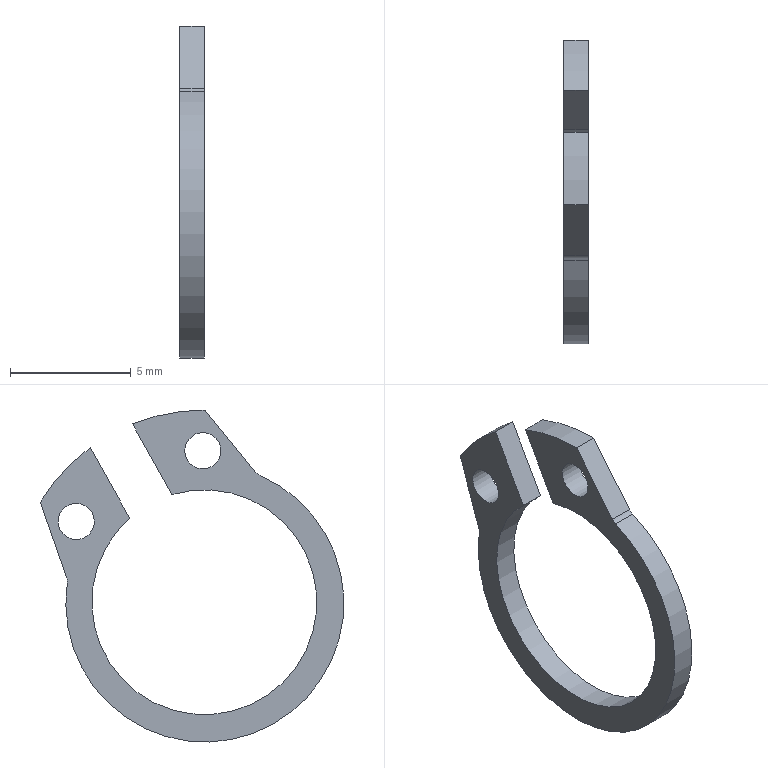Component | NX | RETAINING_RING | 1 solid | 14 faces | box 1 x 12.55 x 13.73 mm | volume 46 mm3 | cylinder 8 | plane 6 | commonest cylinder face diameters 15.9 x2 1.5 x2 1 x2 11.5 x1 9.3 x1
STEP:
#1=CARTESIAN_POINT('',(0.,0.,0.));
#2=DIRECTION('',(0.,0.,1.));
#3=DIRECTION('',(1.,0.,0.));
#4=AXIS2_PLACEMENT_3D('',#1,#2,#3);
#5=CARTESIAN_POINT('',(19.707,5.692,-145.299));
#6=VERTEX_POINT('',#5);
#7=CARTESIAN_POINT('',(19.707,-2.293,-140.838));
#8=VERTEX_POINT('',#7);
#9=CARTESIAN_POINT('',(19.707,0.,-146.111));
#10=DIRECTION('',(-1.,0.,0.));
#11=DIRECTION('',(0.,-0.873,0.4877));
#12=AXIS2_PLACEMENT_3D('',#9,#10,#11);
#13=CIRCLE('',#12,5.75);
#14=CARTESIAN_POINT('',(19.707,0.,-146.111));
#15=DIRECTION('',(-1.,0.,0.));
#16=DIRECTION('',(0.,0.873,-0.4877));
#17=AXIS2_PLACEMENT_3D('',#14,#15,#16);
#18=CYLINDRICAL_SURFACE('',#17,5.75);
#19=CARTESIAN_POINT('',(-3.142,0.));
#20=DIRECTION('',(1.,0.));
#21=VECTOR('',#20,1.);
#22=LINE('',#19,#21);
#23=(GEOMETRIC_REPRESENTATION_CONTEXT(2)PARAMETRIC_REPRESENTATION_CONTEXT()REPRESENTATION_CONTEXT('',''));
#24=DEFINITIONAL_REPRESENTATION('',(#22),#23);
#25=PCURVE('',#18,#24);
#26=CARTESIAN_POINT('',(19.707,0.,-146.111));
#27=DIRECTION('',(-1.,0.,0.));
#28=DIRECTION('',(0.,0.873,-0.4877));
#29=AXIS2_PLACEMENT_3D('',#26,#27,#28);
#30=PLANE('',#29);
#31=CARTESIAN_POINT('',(0.,0.));
#32=DIRECTION('',(-1.,0.));
#33=AXIS2_PLACEMENT_2D('',#31,#32);
#34=CIRCLE('',#33,5.75);
#35=(GEOMETRIC_REPRESENTATION_CONTEXT(2)PARAMETRIC_REPRESENTATION_CONTEXT()REPRESENTATION_CONTEXT('',''));
#36=DEFINITIONAL_REPRESENTATION('',(#34),#35);
#37=PCURVE('',#30,#36);
#38=SURFACE_CURVE('',#13,(#25,#37),.PCURVE_S1.);
#39=EDGE_CURVE('',#6,#8,#38,.T.);
#40=ORIENTED_EDGE('',*,*,#39,.T.);
#41=CARTESIAN_POINT('',(18.707,-2.293,-140.838));
#42=VERTEX_POINT('',#41);
#43=CARTESIAN_POINT('',(19.707,-2.293,-140.838));
#44=DIRECTION('',(-1.,0.,0.));
#45=VECTOR('',#44,1.);
#46=LINE('',#43,#45);
#47=CARTESIAN_POINT('',(3.793,0.));
#48=DIRECTION('',(0.,1.));
#49=VECTOR('',#48,1.);
#50=LINE('',#47,#49);
#51=(GEOMETRIC_REPRESENTATION_CONTEXT(2)PARAMETRIC_REPRESENTATION_CONTEXT()REPRESENTATION_CONTEXT('',''));
#52=DEFINITIONAL_REPRESENTATION('',(#50),#51);
#53=PCURVE('',#18,#52);
#54=CARTESIAN_POINT('',(19.707,-2.492,-140.38));
#55=DIRECTION('',(-1.,0.,0.));
#56=DIRECTION('',(0.,0.873,-0.4877));
#57=AXIS2_PLACEMENT_3D('',#54,#55,#56);
#58=CYLINDRICAL_SURFACE('',#57,0.5);
#59=CARTESIAN_POINT('',(0.6512,0.));
#60=DIRECTION('',(0.,1.));
#61=VECTOR('',#60,1.);
#62=LINE('',#59,#61);
#63=(GEOMETRIC_REPRESENTATION_CONTEXT(2)PARAMETRIC_REPRESENTATION_CONTEXT()REPRESENTATION_CONTEXT('',''));
#64=DEFINITIONAL_REPRESENTATION('',(#62),#63);
#65=PCURVE('',#58,#64);
#66=SURFACE_CURVE('',#46,(#53,#65),.PCURVE_S1.);
#67=EDGE_CURVE('',#8,#42,#66,.T.);
#68=ORIENTED_EDGE('',*,*,#67,.T.);
#69=CARTESIAN_POINT('',(18.707,5.692,-145.299));
#70=VERTEX_POINT('',#69);
#71=CARTESIAN_POINT('',(18.707,0.,-146.111));
#72=DIRECTION('',(-1.,0.,0.));
#73=DIRECTION('',(0.,-0.873,0.4877));
#74=AXIS2_PLACEMENT_3D('',#71,#72,#73);
#75=CIRCLE('',#74,5.75);
#76=CARTESIAN_POINT('',(-3.142,1.));
#77=DIRECTION('',(1.,0.));
#78=VECTOR('',#77,1.);
#79=LINE('',#76,#78);
#80=(GEOMETRIC_REPRESENTATION_CONTEXT(2)PARAMETRIC_REPRESENTATION_CONTEXT()REPRESENTATION_CONTEXT('',''));
#81=DEFINITIONAL_REPRESENTATION('',(#79),#80);
#82=PCURVE('',#18,#81);
#83=CARTESIAN_POINT('',(18.707,0.,-146.111));
#84=DIRECTION('',(-1.,0.,0.));
#85=DIRECTION('',(0.,0.873,-0.4877));
#86=AXIS2_PLACEMENT_3D('',#83,#84,#85);
#87=PLANE('',#86);
#88=CARTESIAN_POINT('',(0.,0.));
#89=DIRECTION('',(-1.,0.));
#90=AXIS2_PLACEMENT_2D('',#88,#89);
#91=CIRCLE('',#90,5.75);
#92=(GEOMETRIC_REPRESENTATION_CONTEXT(2)PARAMETRIC_REPRESENTATION_CONTEXT()REPRESENTATION_CONTEXT('',''));
#93=DEFINITIONAL_REPRESENTATION('',(#91),#92);
#94=PCURVE('',#87,#93);
#95=SURFACE_CURVE('',#75,(#82,#94),.PCURVE_S1.);
#96=EDGE_CURVE('',#70,#42,#95,.T.);
#97=ORIENTED_EDGE('',*,*,#96,.F.);
#98=CARTESIAN_POINT('',(19.707,5.692,-145.299));
#99=DIRECTION('',(1.,0.,0.));
#100=VECTOR('',#99,1.);
#101=LINE('',#98,#100);
#102=CARTESIAN_POINT('',(-0.6512,0.));
#103=DIRECTION('',(0.,-1.));
#104=VECTOR('',#103,1.);
#105=LINE('',#102,#104);
#106=(GEOMETRIC_REPRESENTATION_CONTEXT(2)PARAMETRIC_REPRESENTATION_CONTEXT()REPRESENTATION_CONTEXT('',''));
#107=DEFINITIONAL_REPRESENTATION('',(#105),#106);
#108=PCURVE('',#18,#107);
#109=CARTESIAN_POINT('',(19.707,6.187,-145.228));
#110=DIRECTION('',(-1.,0.,0.));
#111=DIRECTION('',(0.,0.873,-0.4877));
#112=AXIS2_PLACEMENT_3D('',#109,#110,#111);
#113=CYLINDRICAL_SURFACE('',#112,0.5);
#114=CARTESIAN_POINT('',(2.49,0.));
#115=DIRECTION('',(0.,-1.));
#116=VECTOR('',#115,1.);
#117=LINE('',#114,#116);
#118=(GEOMETRIC_REPRESENTATION_CONTEXT(2)PARAMETRIC_REPRESENTATION_CONTEXT()REPRESENTATION_CONTEXT('',''));
#119=DEFINITIONAL_REPRESENTATION('',(#117),#118);
#120=PCURVE('',#113,#119);
#121=SURFACE_CURVE('',#101,(#108,#120),.PCURVE_S1.);
#122=EDGE_CURVE('',#70,#6,#121,.T.);
#123=ORIENTED_EDGE('',*,*,#122,.T.);
#124=EDGE_LOOP('',(#40,#68,#97,#123));
#125=FACE_BOUND('',#124,.T.);
#126=ADVANCED_FACE('',(#125),#18,.T.);
#127=CARTESIAN_POINT('',(18.707,-2.105,-140.696));
#128=VERTEX_POINT('',#127);
#129=CARTESIAN_POINT('',(18.707,-0.01008,-138.126));
#130=VERTEX_POINT('',#129);
#131=CARTESIAN_POINT('',(18.707,-2.183,-140.792));
#132=DIRECTION('',(0.,0.6319,0.7751));
#133=VECTOR('',#132,1.);
#134=LINE('',#131,#133);
#135=CARTESIAN_POINT('',(19.707,-2.183,-140.792));
#136=DIRECTION('',(0.,-0.7751,0.6319));
#137=DIRECTION('',(0.,-0.6319,-0.7751));
#138=AXIS2_PLACEMENT_3D('',#135,#136,#137);
#139=PLANE('',#138);
#140=CARTESIAN_POINT('',(0.,-1.));
#141=DIRECTION('',(-1.,0.));
#142=VECTOR('',#141,1.);
#143=LINE('',#140,#142);
#144=(GEOMETRIC_REPRESENTATION_CONTEXT(2)PARAMETRIC_REPRESENTATION_CONTEXT()REPRESENTATION_CONTEXT('',''));
#145=DEFINITIONAL_REPRESENTATION('',(#143),#144);
#146=PCURVE('',#139,#145);
#147=CARTESIAN_POINT('',(-4.5,-3.579));
#148=DIRECTION('',(0.1736,-0.9848));
#149=VECTOR('',#148,1.);
#150=LINE('',#147,#149);
#151=(GEOMETRIC_REPRESENTATION_CONTEXT(2)PARAMETRIC_REPRESENTATION_CONTEXT()REPRESENTATION_CONTEXT('',''));
#152=DEFINITIONAL_REPRESENTATION('',(#150),#151);
#153=PCURVE('',#87,#152);
#154=SURFACE_CURVE('',#134,(#146,#153),.PCURVE_S1.);
#155=EDGE_CURVE('',#128,#130,#154,.T.);
#156=ORIENTED_EDGE('',*,*,#155,.F.);
#157=CARTESIAN_POINT('',(19.707,-2.105,-140.696));
#158=VERTEX_POINT('',#157);
#159=CARTESIAN_POINT('',(19.707,-2.105,-140.696));
#160=DIRECTION('',(1.,0.,0.));
#161=VECTOR('',#160,1.);
#162=LINE('',#159,#161);
#163=CARTESIAN_POINT('',(-0.1242,0.));
#164=DIRECTION('',(0.,1.));
#165=VECTOR('',#164,1.);
#166=LINE('',#163,#165);
#167=(GEOMETRIC_REPRESENTATION_CONTEXT(2)PARAMETRIC_REPRESENTATION_CONTEXT()REPRESENTATION_CONTEXT('',''));
#168=DEFINITIONAL_REPRESENTATION('',(#166),#167);
#169=PCURVE('',#139,#168);
#170=CARTESIAN_POINT('',(0.1745,0.));
#171=DIRECTION('',(0.,-1.));
#172=VECTOR('',#171,1.);
#173=LINE('',#170,#172);
#174=(GEOMETRIC_REPRESENTATION_CONTEXT(2)PARAMETRIC_REPRESENTATION_CONTEXT()REPRESENTATION_CONTEXT('',''));
#175=DEFINITIONAL_REPRESENTATION('',(#173),#174);
#176=PCURVE('',#58,#175);
#177=SURFACE_CURVE('',#162,(#169,#176),.PCURVE_S1.);
#178=EDGE_CURVE('',#128,#158,#177,.T.);
#179=ORIENTED_EDGE('',*,*,#178,.T.);
#180=CARTESIAN_POINT('',(19.707,-0.01008,-138.126));
#181=VERTEX_POINT('',#180);
#182=CARTESIAN_POINT('',(19.707,-2.183,-140.792));
#183=DIRECTION('',(0.,0.6319,0.7751));
#184=VECTOR('',#183,1.);
#185=LINE('',#182,#184);
#186=CARTESIAN_POINT('',(0.,0.));
#187=DIRECTION('',(-1.,0.));
#188=VECTOR('',#187,1.);
#189=LINE('',#186,#188);
#190=(GEOMETRIC_REPRESENTATION_CONTEXT(2)PARAMETRIC_REPRESENTATION_CONTEXT()REPRESENTATION_CONTEXT('',''));
#191=DEFINITIONAL_REPRESENTATION('',(#189),#190);
#192=PCURVE('',#139,#191);
#193=CARTESIAN_POINT('',(-4.5,-3.579));
#194=DIRECTION('',(0.1736,-0.9848));
#195=VECTOR('',#194,1.);
#196=LINE('',#193,#195);
#197=(GEOMETRIC_REPRESENTATION_CONTEXT(2)PARAMETRIC_REPRESENTATION_CONTEXT()REPRESENTATION_CONTEXT('',''));
#198=DEFINITIONAL_REPRESENTATION('',(#196),#197);
#199=PCURVE('',#30,#198);
#200=SURFACE_CURVE('',#185,(#192,#199),.PCURVE_S1.);
#201=EDGE_CURVE('',#158,#181,#200,.T.);
#202=ORIENTED_EDGE('',*,*,#201,.T.);
#203=CARTESIAN_POINT('',(19.707,-0.01008,-138.126));
#204=DIRECTION('',(-1.,0.,0.));
#205=VECTOR('',#204,1.);
#206=LINE('',#203,#205);
#207=CARTESIAN_POINT('',(-3.439,0.));
#208=DIRECTION('',(0.,-1.));
#209=VECTOR('',#208,1.);
#210=LINE('',#207,#209);
#211=(GEOMETRIC_REPRESENTATION_CONTEXT(2)PARAMETRIC_REPRESENTATION_CONTEXT()REPRESENTATION_CONTEXT('',''));
#212=DEFINITIONAL_REPRESENTATION('',(#210),#211);
#213=PCURVE('',#139,#212);
#214=CARTESIAN_POINT('',(19.707,0.01951,-146.076));
#215=DIRECTION('',(-1.,0.,0.));
#216=DIRECTION('',(0.,0.873,-0.4877));
#217=AXIS2_PLACEMENT_3D('',#214,#215,#216);
#218=CYLINDRICAL_SURFACE('',#217,7.95);
#219=CARTESIAN_POINT('',(4.199,0.));
#220=DIRECTION('',(0.,1.));
#221=VECTOR('',#220,1.);
#222=LINE('',#219,#221);
#223=(GEOMETRIC_REPRESENTATION_CONTEXT(2)PARAMETRIC_REPRESENTATION_CONTEXT()REPRESENTATION_CONTEXT('',''));
#224=DEFINITIONAL_REPRESENTATION('',(#222),#223);
#225=PCURVE('',#218,#224);
#226=SURFACE_CURVE('',#206,(#213,#225),.PCURVE_S1.);
#227=EDGE_CURVE('',#181,#130,#226,.T.);
#228=ORIENTED_EDGE('',*,*,#227,.T.);
#229=EDGE_LOOP('',(#156,#179,#202,#228));
#230=FACE_BOUND('',#229,.T.);
#231=ADVANCED_FACE('',(#230),#139,.T.);
#232=CARTESIAN_POINT('',(18.707,2.993,-138.703));
#233=VERTEX_POINT('',#232);
#234=CARTESIAN_POINT('',(18.707,0.01951,-146.076));
#235=DIRECTION('',(-1.,0.,0.));
#236=DIRECTION('',(0.,-0.873,0.4877));
#237=AXIS2_PLACEMENT_3D('',#234,#235,#236);
#238=CIRCLE('',#237,7.95);
#239=CARTESIAN_POINT('',(3.142,1.));
#240=DIRECTION('',(1.,0.));
#241=VECTOR('',#240,1.);
#242=LINE('',#239,#241);
#243=(GEOMETRIC_REPRESENTATION_CONTEXT(2)PARAMETRIC_REPRESENTATION_CONTEXT()REPRESENTATION_CONTEXT('',''));
#244=DEFINITIONAL_REPRESENTATION('',(#242),#243);
#245=PCURVE('',#218,#244);
#246=CARTESIAN_POINT('',(-0.,-0.04));
#247=DIRECTION('',(-1.,0.));
#248=AXIS2_PLACEMENT_2D('',#246,#247);
#249=CIRCLE('',#248,7.95);
#250=(GEOMETRIC_REPRESENTATION_CONTEXT(2)PARAMETRIC_REPRESENTATION_CONTEXT()REPRESENTATION_CONTEXT('',''));
#251=DEFINITIONAL_REPRESENTATION('',(#249),#250);
#252=PCURVE('',#87,#251);
#253=SURFACE_CURVE('',#238,(#245,#252),.PCURVE_S1.);
#254=EDGE_CURVE('',#130,#233,#253,.T.);
#255=ORIENTED_EDGE('',*,*,#254,.F.);
#256=ORIENTED_EDGE('',*,*,#227,.F.);
#257=CARTESIAN_POINT('',(19.707,2.993,-138.703));
#258=VERTEX_POINT('',#257);
#259=CARTESIAN_POINT('',(19.707,0.01951,-146.076));
#260=DIRECTION('',(-1.,0.,0.));
#261=DIRECTION('',(0.,-0.873,0.4877));
#262=AXIS2_PLACEMENT_3D('',#259,#260,#261);
#263=CIRCLE('',#262,7.95);
#264=CARTESIAN_POINT('',(3.142,0.));
#265=DIRECTION('',(1.,0.));
#266=VECTOR('',#265,1.);
#267=LINE('',#264,#266);
#268=(GEOMETRIC_REPRESENTATION_CONTEXT(2)PARAMETRIC_REPRESENTATION_CONTEXT()REPRESENTATION_CONTEXT('',''));
#269=DEFINITIONAL_REPRESENTATION('',(#267),#268);
#270=PCURVE('',#218,#269);
#271=CARTESIAN_POINT('',(-0.,-0.04));
#272=DIRECTION('',(-1.,0.));
#273=AXIS2_PLACEMENT_2D('',#271,#272);
#274=CIRCLE('',#273,7.95);
#275=(GEOMETRIC_REPRESENTATION_CONTEXT(2)PARAMETRIC_REPRESENTATION_CONTEXT()REPRESENTATION_CONTEXT('',''));
#276=DEFINITIONAL_REPRESENTATION('',(#274),#275);
#277=PCURVE('',#30,#276);
#278=SURFACE_CURVE('',#263,(#270,#277),.PCURVE_S1.);
#279=EDGE_CURVE('',#181,#258,#278,.T.);
#280=ORIENTED_EDGE('',*,*,#279,.T.);
#281=CARTESIAN_POINT('',(19.707,2.993,-138.703));
#282=DIRECTION('',(-1.,0.,0.));
#283=VECTOR('',#282,1.);
#284=LINE('',#281,#283);
#285=CARTESIAN_POINT('',(4.586,0.));
#286=DIRECTION('',(0.,1.));
#287=VECTOR('',#286,1.);
#288=LINE('',#285,#287);
#289=(GEOMETRIC_REPRESENTATION_CONTEXT(2)PARAMETRIC_REPRESENTATION_CONTEXT()REPRESENTATION_CONTEXT('',''));
#290=DEFINITIONAL_REPRESENTATION('',(#288),#289);
#291=PCURVE('',#218,#290);
#292=CARTESIAN_POINT('',(19.707,2.993,-138.703));
#293=DIRECTION('',(0.,0.873,-0.4877));
#294=DIRECTION('',(0.,0.4877,0.873));
#295=AXIS2_PLACEMENT_3D('',#292,#293,#294);
#296=PLANE('',#295);
#297=CARTESIAN_POINT('',(0.,0.));
#298=DIRECTION('',(0.,-1.));
#299=VECTOR('',#298,1.);
#300=LINE('',#297,#299);
#301=(GEOMETRIC_REPRESENTATION_CONTEXT(2)PARAMETRIC_REPRESENTATION_CONTEXT()REPRESENTATION_CONTEXT('',''));
#302=DEFINITIONAL_REPRESENTATION('',(#300),#301);
#303=PCURVE('',#296,#302);
#304=SURFACE_CURVE('',#284,(#291,#303),.PCURVE_S1.);
#305=EDGE_CURVE('',#258,#233,#304,.T.);
#306=ORIENTED_EDGE('',*,*,#305,.T.);
#307=EDGE_LOOP('',(#255,#256,#280,#306));
#308=FACE_BOUND('',#307,.T.);
#309=ADVANCED_FACE('',(#308),#218,.T.);
#310=CARTESIAN_POINT('',(18.707,1.361,-141.624));
#311=VERTEX_POINT('',#310);
#312=CARTESIAN_POINT('',(18.707,2.993,-138.703));
#313=DIRECTION('',(0.,-0.4877,-0.873));
#314=VECTOR('',#313,1.);
#315=LINE('',#312,#314);
#316=CARTESIAN_POINT('',(0.,-1.));
#317=DIRECTION('',(-1.,0.));
#318=VECTOR('',#317,1.);
#319=LINE('',#316,#318);
#320=(GEOMETRIC_REPRESENTATION_CONTEXT(2)PARAMETRIC_REPRESENTATION_CONTEXT()REPRESENTATION_CONTEXT('',''));
#321=DEFINITIONAL_REPRESENTATION('',(#319),#320);
#322=PCURVE('',#296,#321);
#323=CARTESIAN_POINT('',(-1.,-7.927));
#324=DIRECTION('',(0.,1.));
#325=VECTOR('',#324,1.);
#326=LINE('',#323,#325);
#327=(GEOMETRIC_REPRESENTATION_CONTEXT(2)PARAMETRIC_REPRESENTATION_CONTEXT()REPRESENTATION_CONTEXT('',''));
#328=DEFINITIONAL_REPRESENTATION('',(#326),#327);
#329=PCURVE('',#87,#328);
#330=SURFACE_CURVE('',#315,(#322,#329),.PCURVE_S1.);
#331=EDGE_CURVE('',#233,#311,#330,.T.);
#332=ORIENTED_EDGE('',*,*,#331,.F.);
#333=ORIENTED_EDGE('',*,*,#305,.F.);
#334=CARTESIAN_POINT('',(19.707,1.361,-141.624));
#335=VERTEX_POINT('',#334);
#336=CARTESIAN_POINT('',(19.707,2.993,-138.703));
#337=DIRECTION('',(0.,-0.4877,-0.873));
#338=VECTOR('',#337,1.);
#339=LINE('',#336,#338);
#340=CARTESIAN_POINT('',(0.,0.));
#341=DIRECTION('',(-1.,0.));
#342=VECTOR('',#341,1.);
#343=LINE('',#340,#342);
#344=(GEOMETRIC_REPRESENTATION_CONTEXT(2)PARAMETRIC_REPRESENTATION_CONTEXT()REPRESENTATION_CONTEXT('',''));
#345=DEFINITIONAL_REPRESENTATION('',(#343),#344);
#346=PCURVE('',#296,#345);
#347=CARTESIAN_POINT('',(-1.,-7.927));
#348=DIRECTION('',(0.,1.));
#349=VECTOR('',#348,1.);
#350=LINE('',#347,#349);
#351=(GEOMETRIC_REPRESENTATION_CONTEXT(2)PARAMETRIC_REPRESENTATION_CONTEXT()REPRESENTATION_CONTEXT('',''));
#352=DEFINITIONAL_REPRESENTATION('',(#350),#351);
#353=PCURVE('',#30,#352);
#354=SURFACE_CURVE('',#339,(#346,#353),.PCURVE_S1.);
#355=EDGE_CURVE('',#258,#335,#354,.T.);
#356=ORIENTED_EDGE('',*,*,#355,.T.);
#357=CARTESIAN_POINT('',(19.707,1.361,-141.624));
#358=DIRECTION('',(-1.,0.,0.));
#359=VECTOR('',#358,1.);
#360=LINE('',#357,#359);
#361=CARTESIAN_POINT('',(-3.346,0.));
#362=DIRECTION('',(0.,-1.));
#363=VECTOR('',#362,1.);
#364=LINE('',#361,#363);
#365=(GEOMETRIC_REPRESENTATION_CONTEXT(2)PARAMETRIC_REPRESENTATION_CONTEXT()REPRESENTATION_CONTEXT('',''));
#366=DEFINITIONAL_REPRESENTATION('',(#364),#365);
#367=PCURVE('',#296,#366);
#368=CARTESIAN_POINT('',(19.707,0.01951,-146.076));
#369=DIRECTION('',(-1.,0.,0.));
#370=DIRECTION('',(0.,0.873,-0.4877));
#371=AXIS2_PLACEMENT_3D('',#368,#369,#370);
#372=CYLINDRICAL_SURFACE('',#371,4.65);
#373=CARTESIAN_POINT('',(4.496,0.));
#374=DIRECTION('',(0.,1.));
#375=VECTOR('',#374,1.);
#376=LINE('',#373,#375);
#377=(GEOMETRIC_REPRESENTATION_CONTEXT(2)PARAMETRIC_REPRESENTATION_CONTEXT()REPRESENTATION_CONTEXT('',''));
#378=DEFINITIONAL_REPRESENTATION('',(#376),#377);
#379=PCURVE('',#372,#378);
#380=SURFACE_CURVE('',#360,(#367,#379),.PCURVE_S1.);
#381=EDGE_CURVE('',#335,#311,#380,.T.);
#382=ORIENTED_EDGE('',*,*,#381,.T.);
#383=EDGE_LOOP('',(#332,#333,#356,#382));
#384=FACE_BOUND('',#383,.T.);
#385=ADVANCED_FACE('',(#384),#296,.T.);
#386=CARTESIAN_POINT('',(19.707,3.107,-142.599));
#387=VERTEX_POINT('',#386);
#388=CARTESIAN_POINT('',(18.707,3.107,-142.599));
#389=VERTEX_POINT('',#388);
#390=CARTESIAN_POINT('',(19.707,3.107,-142.599));
#391=DIRECTION('',(-1.,0.,0.));
#392=VECTOR('',#391,1.);
#393=LINE('',#390,#392);
#394=CARTESIAN_POINT('',(-1.354,0.));
#395=DIRECTION('',(0.,1.));
#396=VECTOR('',#395,1.);
#397=LINE('',#394,#396);
#398=(GEOMETRIC_REPRESENTATION_CONTEXT(2)PARAMETRIC_REPRESENTATION_CONTEXT()REPRESENTATION_CONTEXT('',''));
#399=DEFINITIONAL_REPRESENTATION('',(#397),#398);
#400=PCURVE('',#372,#399);
#401=CARTESIAN_POINT('',(19.707,3.107,-142.599));
#402=DIRECTION('',(0.,-0.873,0.4877));
#403=DIRECTION('',(0.,-0.4877,-0.873));
#404=AXIS2_PLACEMENT_3D('',#401,#402,#403);
#405=PLANE('',#404);
#406=CARTESIAN_POINT('',(0.,0.));
#407=DIRECTION('',(0.,-1.));
#408=VECTOR('',#407,1.);
#409=LINE('',#406,#408);
#410=(GEOMETRIC_REPRESENTATION_CONTEXT(2)PARAMETRIC_REPRESENTATION_CONTEXT()REPRESENTATION_CONTEXT('',''));
#411=DEFINITIONAL_REPRESENTATION('',(#409),#410);
#412=PCURVE('',#405,#411);
#413=SURFACE_CURVE('',#393,(#400,#412),.PCURVE_S1.);
#414=EDGE_CURVE('',#387,#389,#413,.T.);
#415=ORIENTED_EDGE('',*,*,#414,.F.);
#416=CARTESIAN_POINT('',(19.707,0.01951,-146.076));
#417=DIRECTION('',(1.,0.,0.));
#418=DIRECTION('',(0.,-0.873,0.4877));
#419=AXIS2_PLACEMENT_3D('',#416,#417,#418);
#420=CIRCLE('',#419,4.65);
#421=CARTESIAN_POINT('',(9.425,0.));
#422=DIRECTION('',(-1.,0.));
#423=VECTOR('',#422,1.);
#424=LINE('',#421,#423);
#425=(GEOMETRIC_REPRESENTATION_CONTEXT(2)PARAMETRIC_REPRESENTATION_CONTEXT()REPRESENTATION_CONTEXT('',''));
#426=DEFINITIONAL_REPRESENTATION('',(#424),#425);
#427=PCURVE('',#372,#426);
#428=CARTESIAN_POINT('',(-4.65,-0.04));
#429=CARTESIAN_POINT('',(-4.65,8.014));
#430=CARTESIAN_POINT('',(2.325,3.987));
#431=CARTESIAN_POINT('',(9.3,-0.04));
#432=CARTESIAN_POINT('',(2.325,-4.067));
#433=CARTESIAN_POINT('',(-4.65,-8.094));
#434=CARTESIAN_POINT('',(-4.65,-0.04));
#435=(BOUNDED_CURVE()B_SPLINE_CURVE(2,(#428,#429,#430,#431,#432,#433,#434),.UNSPECIFIED.,.T.,.F.)B_SPLINE_CURVE_WITH_KNOTS((1,2,2,2,2,1),(-2.094,0.,2.094,4.189,6.283,8.378),.UNSPECIFIED.)CURVE()GEOMETRIC_REPRESENTATION_ITEM()RATIONAL_B_SPLINE_CURVE((1.,0.5,1.,0.5,1.,0.5,1.))REPRESENTATION_ITEM(''));
#436=(GEOMETRIC_REPRESENTATION_CONTEXT(2)PARAMETRIC_REPRESENTATION_CONTEXT()REPRESENTATION_CONTEXT('',''));
#437=DEFINITIONAL_REPRESENTATION('',(#435),#436);
#438=PCURVE('',#30,#437);
#439=SURFACE_CURVE('',#420,(#427,#438),.PCURVE_S1.);
#440=EDGE_CURVE('',#335,#387,#439,.T.);
#441=ORIENTED_EDGE('',*,*,#440,.F.);
#442=ORIENTED_EDGE('',*,*,#381,.T.);
#443=CARTESIAN_POINT('',(18.707,0.01951,-146.076));
#444=DIRECTION('',(1.,0.,0.));
#445=DIRECTION('',(0.,-0.873,0.4877));
#446=AXIS2_PLACEMENT_3D('',#443,#444,#445);
#447=CIRCLE('',#446,4.65);
#448=CARTESIAN_POINT('',(9.425,1.));
#449=DIRECTION('',(-1.,0.));
#450=VECTOR('',#449,1.);
#451=LINE('',#448,#450);
#452=(GEOMETRIC_REPRESENTATION_CONTEXT(2)PARAMETRIC_REPRESENTATION_CONTEXT()REPRESENTATION_CONTEXT('',''));
#453=DEFINITIONAL_REPRESENTATION('',(#451),#452);
#454=PCURVE('',#372,#453);
#455=CARTESIAN_POINT('',(-4.65,-0.04));
#456=CARTESIAN_POINT('',(-4.65,8.014));
#457=CARTESIAN_POINT('',(2.325,3.987));
#458=CARTESIAN_POINT('',(9.3,-0.04));
#459=CARTESIAN_POINT('',(2.325,-4.067));
#460=CARTESIAN_POINT('',(-4.65,-8.094));
#461=CARTESIAN_POINT('',(-4.65,-0.04));
#462=(BOUNDED_CURVE()B_SPLINE_CURVE(2,(#455,#456,#457,#458,#459,#460,#461),.UNSPECIFIED.,.T.,.F.)B_SPLINE_CURVE_WITH_KNOTS((1,2,2,2,2,1),(-2.094,0.,2.094,4.189,6.283,8.378),.UNSPECIFIED.)CURVE()GEOMETRIC_REPRESENTATION_ITEM()RATIONAL_B_SPLINE_CURVE((1.,0.5,1.,0.5,1.,0.5,1.))REPRESENTATION_ITEM(''));
#463=(GEOMETRIC_REPRESENTATION_CONTEXT(2)PARAMETRIC_REPRESENTATION_CONTEXT()REPRESENTATION_CONTEXT('',''));
#464=DEFINITIONAL_REPRESENTATION('',(#462),#463);
#465=PCURVE('',#87,#464);
#466=SURFACE_CURVE('',#447,(#454,#465),.PCURVE_S1.);
#467=EDGE_CURVE('',#311,#389,#466,.T.);
#468=ORIENTED_EDGE('',*,*,#467,.T.);
#469=EDGE_LOOP('',(#415,#441,#442,#468));
#470=FACE_BOUND('',#469,.F.);
#471=ADVANCED_FACE('',(#470),#372,.F.);
#472=CARTESIAN_POINT('',(18.707,4.739,-139.679));
#473=VERTEX_POINT('',#472);
#474=CARTESIAN_POINT('',(18.707,3.107,-142.599));
#475=DIRECTION('',(0.,0.4877,0.873));
#476=VECTOR('',#475,1.);
#477=LINE('',#474,#476);
#478=CARTESIAN_POINT('',(0.,-1.));
#479=DIRECTION('',(-1.,0.));
#480=VECTOR('',#479,1.);
#481=LINE('',#478,#480);
#482=(GEOMETRIC_REPRESENTATION_CONTEXT(2)PARAMETRIC_REPRESENTATION_CONTEXT()REPRESENTATION_CONTEXT('',''));
#483=DEFINITIONAL_REPRESENTATION('',(#481),#482);
#484=PCURVE('',#405,#483);
#485=CARTESIAN_POINT('',(1.,-4.581));
#486=DIRECTION('',(0.,-1.));
#487=VECTOR('',#486,1.);
#488=LINE('',#485,#487);
#489=(GEOMETRIC_REPRESENTATION_CONTEXT(2)PARAMETRIC_REPRESENTATION_CONTEXT()REPRESENTATION_CONTEXT('',''));
#490=DEFINITIONAL_REPRESENTATION('',(#488),#489);
#491=PCURVE('',#87,#490);
#492=SURFACE_CURVE('',#477,(#484,#491),.PCURVE_S1.);
#493=EDGE_CURVE('',#389,#473,#492,.T.);
#494=ORIENTED_EDGE('',*,*,#493,.F.);
#495=ORIENTED_EDGE('',*,*,#414,.F.);
#496=CARTESIAN_POINT('',(19.707,4.739,-139.679));
#497=VERTEX_POINT('',#496);
#498=CARTESIAN_POINT('',(19.707,3.107,-142.599));
#499=DIRECTION('',(0.,0.4877,0.873));
#500=VECTOR('',#499,1.);
#501=LINE('',#498,#500);
#502=CARTESIAN_POINT('',(0.,0.));
#503=DIRECTION('',(-1.,0.));
#504=VECTOR('',#503,1.);
#505=LINE('',#502,#504);
#506=(GEOMETRIC_REPRESENTATION_CONTEXT(2)PARAMETRIC_REPRESENTATION_CONTEXT()REPRESENTATION_CONTEXT('',''));
#507=DEFINITIONAL_REPRESENTATION('',(#505),#506);
#508=PCURVE('',#405,#507);
#509=CARTESIAN_POINT('',(1.,-4.581));
#510=DIRECTION('',(0.,-1.));
#511=VECTOR('',#510,1.);
#512=LINE('',#509,#511);
#513=(GEOMETRIC_REPRESENTATION_CONTEXT(2)PARAMETRIC_REPRESENTATION_CONTEXT()REPRESENTATION_CONTEXT('',''));
#514=DEFINITIONAL_REPRESENTATION('',(#512),#513);
#515=PCURVE('',#30,#514);
#516=SURFACE_CURVE('',#501,(#508,#515),.PCURVE_S1.);
#517=EDGE_CURVE('',#387,#497,#516,.T.);
#518=ORIENTED_EDGE('',*,*,#517,.T.);
#519=CARTESIAN_POINT('',(19.707,4.739,-139.679));
#520=DIRECTION('',(-1.,0.,0.));
#521=VECTOR('',#520,1.);
#522=LINE('',#519,#521);
#523=CARTESIAN_POINT('',(-3.346,0.));
#524=DIRECTION('',(0.,-1.));
#525=VECTOR('',#524,1.);
#526=LINE('',#523,#525);
#527=(GEOMETRIC_REPRESENTATION_CONTEXT(2)PARAMETRIC_REPRESENTATION_CONTEXT()REPRESENTATION_CONTEXT('',''));
#528=DEFINITIONAL_REPRESENTATION('',(#526),#527);
#529=PCURVE('',#405,#528);
#530=CARTESIAN_POINT('',(19.707,0.01951,-146.076));
#531=DIRECTION('',(-1.,0.,0.));
#532=DIRECTION('',(0.,0.873,-0.4877));
#533=AXIS2_PLACEMENT_3D('',#530,#531,#532);
#534=CYLINDRICAL_SURFACE('',#533,7.95);
#535=CARTESIAN_POINT('',(4.839,0.));
#536=DIRECTION('',(0.,1.));
#537=VECTOR('',#536,1.);
#538=LINE('',#535,#537);
#539=(GEOMETRIC_REPRESENTATION_CONTEXT(2)PARAMETRIC_REPRESENTATION_CONTEXT()REPRESENTATION_CONTEXT('',''));
#540=DEFINITIONAL_REPRESENTATION('',(#538),#539);
#541=PCURVE('',#534,#540);
#542=SURFACE_CURVE('',#522,(#529,#541),.PCURVE_S1.);
#543=EDGE_CURVE('',#497,#473,#542,.T.);
#544=ORIENTED_EDGE('',*,*,#543,.T.);
#545=EDGE_LOOP('',(#494,#495,#518,#544));
#546=FACE_BOUND('',#545,.T.);
#547=ADVANCED_FACE('',(#546),#405,.T.);
#548=CARTESIAN_POINT('',(18.707,6.804,-141.933));
#549=VERTEX_POINT('',#548);
#550=CARTESIAN_POINT('',(18.707,0.01951,-146.076));
#551=DIRECTION('',(-1.,0.,0.));
#552=DIRECTION('',(0.,-0.873,0.4877));
#553=AXIS2_PLACEMENT_3D('',#550,#551,#552);
#554=CIRCLE('',#553,7.95);
#555=CARTESIAN_POINT('',(3.142,1.));
#556=DIRECTION('',(1.,0.));
#557=VECTOR('',#556,1.);
#558=LINE('',#555,#557);
#559=(GEOMETRIC_REPRESENTATION_CONTEXT(2)PARAMETRIC_REPRESENTATION_CONTEXT()REPRESENTATION_CONTEXT('',''));
#560=DEFINITIONAL_REPRESENTATION('',(#558),#559);
#561=PCURVE('',#534,#560);
#562=CARTESIAN_POINT('',(-0.,-0.04));
#563=DIRECTION('',(-1.,0.));
#564=AXIS2_PLACEMENT_2D('',#562,#563);
#565=CIRCLE('',#564,7.95);
#566=(GEOMETRIC_REPRESENTATION_CONTEXT(2)PARAMETRIC_REPRESENTATION_CONTEXT()REPRESENTATION_CONTEXT('',''));
#567=DEFINITIONAL_REPRESENTATION('',(#565),#566);
#568=PCURVE('',#87,#567);
#569=SURFACE_CURVE('',#554,(#561,#568),.PCURVE_S1.);
#570=EDGE_CURVE('',#473,#549,#569,.T.);
#571=ORIENTED_EDGE('',*,*,#570,.F.);
#572=ORIENTED_EDGE('',*,*,#543,.F.);
#573=CARTESIAN_POINT('',(19.707,6.804,-141.933));
#574=VERTEX_POINT('',#573);
#575=CARTESIAN_POINT('',(19.707,0.01951,-146.076));
#576=DIRECTION('',(-1.,0.,0.));
#577=DIRECTION('',(0.,-0.873,0.4877));
#578=AXIS2_PLACEMENT_3D('',#575,#576,#577);
#579=CIRCLE('',#578,7.95);
#580=CARTESIAN_POINT('',(3.142,0.));
#581=DIRECTION('',(1.,0.));
#582=VECTOR('',#581,1.);
#583=LINE('',#580,#582);
#584=(GEOMETRIC_REPRESENTATION_CONTEXT(2)PARAMETRIC_REPRESENTATION_CONTEXT()REPRESENTATION_CONTEXT('',''));
#585=DEFINITIONAL_REPRESENTATION('',(#583),#584);
#586=PCURVE('',#534,#585);
#587=CARTESIAN_POINT('',(-0.,-0.04));
#588=DIRECTION('',(-1.,0.));
#589=AXIS2_PLACEMENT_2D('',#587,#588);
#590=CIRCLE('',#589,7.95);
#591=(GEOMETRIC_REPRESENTATION_CONTEXT(2)PARAMETRIC_REPRESENTATION_CONTEXT()REPRESENTATION_CONTEXT('',''));
#592=DEFINITIONAL_REPRESENTATION('',(#590),#591);
#593=PCURVE('',#30,#592);
#594=SURFACE_CURVE('',#579,(#586,#593),.PCURVE_S1.);
#595=EDGE_CURVE('',#497,#574,#594,.T.);
#596=ORIENTED_EDGE('',*,*,#595,.T.);
#597=CARTESIAN_POINT('',(19.707,6.804,-141.933));
#598=DIRECTION('',(-1.,0.,0.));
#599=VECTOR('',#598,1.);
#600=LINE('',#597,#599);
#601=CARTESIAN_POINT('',(5.226,0.));
#602=DIRECTION('',(0.,1.));
#603=VECTOR('',#602,1.);
#604=LINE('',#601,#603);
#605=(GEOMETRIC_REPRESENTATION_CONTEXT(2)PARAMETRIC_REPRESENTATION_CONTEXT()REPRESENTATION_CONTEXT('',''));
#606=DEFINITIONAL_REPRESENTATION('',(#604),#605);
#607=PCURVE('',#534,#606);
#608=CARTESIAN_POINT('',(19.707,6.804,-141.933));
#609=DIRECTION('',(0.,0.9444,-0.3287));
#610=DIRECTION('',(0.,0.3287,0.9444));
#611=AXIS2_PLACEMENT_3D('',#608,#609,#610);
#612=PLANE('',#611);
#613=CARTESIAN_POINT('',(-0.,0.));
#614=DIRECTION('',(0.,-1.));
#615=VECTOR('',#614,1.);
#616=LINE('',#613,#615);
#617=(GEOMETRIC_REPRESENTATION_CONTEXT(2)PARAMETRIC_REPRESENTATION_CONTEXT()REPRESENTATION_CONTEXT('',''));
#618=DEFINITIONAL_REPRESENTATION('',(#616),#617);
#619=PCURVE('',#612,#618);
#620=SURFACE_CURVE('',#600,(#607,#619),.PCURVE_S1.);
#621=EDGE_CURVE('',#574,#549,#620,.T.);
#622=ORIENTED_EDGE('',*,*,#621,.T.);
#623=EDGE_LOOP('',(#571,#572,#596,#622));
#624=FACE_BOUND('',#623,.T.);
#625=ADVANCED_FACE('',(#624),#534,.T.);
#626=CARTESIAN_POINT('',(19.707,0.7374,-140.177));
#627=VERTEX_POINT('',#626);
#628=CARTESIAN_POINT('',(19.707,0.08267,-139.812));
#629=DIRECTION('',(1.,0.,0.));
#630=DIRECTION('',(0.,0.873,-0.4877));
#631=AXIS2_PLACEMENT_3D('',#628,#629,#630);
#632=CIRCLE('',#631,0.75);
#633=CARTESIAN_POINT('',(19.707,0.08267,-139.812));
#634=DIRECTION('',(-1.,0.,0.));
#635=DIRECTION('',(0.,0.873,-0.4877));
#636=AXIS2_PLACEMENT_3D('',#633,#634,#635);
#637=CYLINDRICAL_SURFACE('',#636,0.75);
#638=CARTESIAN_POINT('',(6.283,0.));
#639=DIRECTION('',(-1.,0.));
#640=VECTOR('',#639,1.);
#641=LINE('',#638,#640);
#642=(GEOMETRIC_REPRESENTATION_CONTEXT(2)PARAMETRIC_REPRESENTATION_CONTEXT()REPRESENTATION_CONTEXT('',''));
#643=DEFINITIONAL_REPRESENTATION('',(#641),#642);
#644=PCURVE('',#637,#643);
#645=CARTESIAN_POINT('',(-2.25,-5.54));
#646=CARTESIAN_POINT('',(-2.25,-6.839));
#647=CARTESIAN_POINT('',(-3.375,-6.19));
#648=CARTESIAN_POINT('',(-4.5,-5.54));
#649=CARTESIAN_POINT('',(-3.375,-4.89));
#650=CARTESIAN_POINT('',(-2.25,-4.241));
#651=CARTESIAN_POINT('',(-2.25,-5.54));
#652=(BOUNDED_CURVE()B_SPLINE_CURVE(2,(#645,#646,#647,#648,#649,#650,#651),.UNSPECIFIED.,.T.,.F.)B_SPLINE_CURVE_WITH_KNOTS((1,2,2,2,2,1),(-2.094,0.,2.094,4.189,6.283,8.378),.UNSPECIFIED.)CURVE()GEOMETRIC_REPRESENTATION_ITEM()RATIONAL_B_SPLINE_CURVE((1.,0.5,1.,0.5,1.,0.5,1.))REPRESENTATION_ITEM(''));
#653=(GEOMETRIC_REPRESENTATION_CONTEXT(2)PARAMETRIC_REPRESENTATION_CONTEXT()REPRESENTATION_CONTEXT('',''));
#654=DEFINITIONAL_REPRESENTATION('',(#652),#653);
#655=PCURVE('',#30,#654);
#656=SURFACE_CURVE('',#632,(#644,#655),.PCURVE_S1.);
#657=EDGE_CURVE('',#627,#627,#656,.T.);
#658=ORIENTED_EDGE('',*,*,#657,.F.);
#659=CARTESIAN_POINT('',(18.707,0.7374,-140.177));
#660=VERTEX_POINT('',#659);
#661=CARTESIAN_POINT('',(19.707,0.7374,-140.177));
#662=CARTESIAN_POINT('',(18.707,0.7374,-140.177));
#663=B_SPLINE_CURVE_WITH_KNOTS('',1,(#661,#662),.UNSPECIFIED.,.F.,.F.,(2,2),(0.,1.),.PIECEWISE_BEZIER_KNOTS.);
#664=CARTESIAN_POINT('',(6.283,0.));
#665=DIRECTION('',(0.,1.));
#666=VECTOR('',#665,1.);
#667=LINE('',#664,#666);
#668=(GEOMETRIC_REPRESENTATION_CONTEXT(2)PARAMETRIC_REPRESENTATION_CONTEXT()REPRESENTATION_CONTEXT('',''));
#669=DEFINITIONAL_REPRESENTATION('',(#667),#668);
#670=PCURVE('',#637,#669);
#671=CARTESIAN_POINT('',(0.,0.));
#672=DIRECTION('',(0.,1.));
#673=VECTOR('',#672,1.);
#674=LINE('',#671,#673);
#675=(GEOMETRIC_REPRESENTATION_CONTEXT(2)PARAMETRIC_REPRESENTATION_CONTEXT()REPRESENTATION_CONTEXT('',''));
#676=DEFINITIONAL_REPRESENTATION('',(#674),#675);
#677=PCURVE('',#637,#676);
#678=SEAM_CURVE('',#663,(#670,#677),.PCURVE_S1.);
#679=EDGE_CURVE('',#627,#660,#678,.T.);
#680=ORIENTED_EDGE('',*,*,#679,.T.);
#681=CARTESIAN_POINT('',(18.707,0.08267,-139.812));
#682=DIRECTION('',(1.,0.,0.));
#683=DIRECTION('',(0.,0.873,-0.4877));
#684=AXIS2_PLACEMENT_3D('',#681,#682,#683);
#685=CIRCLE('',#684,0.75);
#686=CARTESIAN_POINT('',(6.283,1.));
#687=DIRECTION('',(-1.,0.));
#688=VECTOR('',#687,1.);
#689=LINE('',#686,#688);
#690=(GEOMETRIC_REPRESENTATION_CONTEXT(2)PARAMETRIC_REPRESENTATION_CONTEXT()REPRESENTATION_CONTEXT('',''));
#691=DEFINITIONAL_REPRESENTATION('',(#689),#690);
#692=PCURVE('',#637,#691);
#693=CARTESIAN_POINT('',(-2.25,-5.54));
#694=CARTESIAN_POINT('',(-2.25,-6.839));
#695=CARTESIAN_POINT('',(-3.375,-6.19));
#696=CARTESIAN_POINT('',(-4.5,-5.54));
#697=CARTESIAN_POINT('',(-3.375,-4.89));
#698=CARTESIAN_POINT('',(-2.25,-4.241));
#699=CARTESIAN_POINT('',(-2.25,-5.54));
#700=(BOUNDED_CURVE()B_SPLINE_CURVE(2,(#693,#694,#695,#696,#697,#698,#699),.UNSPECIFIED.,.T.,.F.)B_SPLINE_CURVE_WITH_KNOTS((1,2,2,2,2,1),(-2.094,0.,2.094,4.189,6.283,8.378),.UNSPECIFIED.)CURVE()GEOMETRIC_REPRESENTATION_ITEM()RATIONAL_B_SPLINE_CURVE((1.,0.5,1.,0.5,1.,0.5,1.))REPRESENTATION_ITEM(''));
#701=(GEOMETRIC_REPRESENTATION_CONTEXT(2)PARAMETRIC_REPRESENTATION_CONTEXT()REPRESENTATION_CONTEXT('',''));
#702=DEFINITIONAL_REPRESENTATION('',(#700),#701);
#703=PCURVE('',#87,#702);
#704=SURFACE_CURVE('',#685,(#692,#703),.PCURVE_S1.);
#705=EDGE_CURVE('',#660,#660,#704,.T.);
#706=ORIENTED_EDGE('',*,*,#705,.T.);
#707=ORIENTED_EDGE('',*,*,#679,.F.);
#708=EDGE_LOOP('',(#658,#680,#706,#707));
#709=FACE_BOUND('',#708,.F.);
#710=ADVANCED_FACE('',(#709),#637,.F.);
#711=CARTESIAN_POINT('',(19.707,5.715,-145.064));
#712=VERTEX_POINT('',#711);
#713=CARTESIAN_POINT('',(19.707,6.804,-141.933));
#714=DIRECTION('',(0.,-0.3287,-0.9444));
#715=VECTOR('',#714,1.);
#716=LINE('',#713,#715);
#717=CARTESIAN_POINT('',(0.,0.));
#718=DIRECTION('',(-1.,0.));
#719=VECTOR('',#718,1.);
#720=LINE('',#717,#719);
#721=(GEOMETRIC_REPRESENTATION_CONTEXT(2)PARAMETRIC_REPRESENTATION_CONTEXT()REPRESENTATION_CONTEXT('',''));
#722=DEFINITIONAL_REPRESENTATION('',(#720),#721);
#723=PCURVE('',#612,#722);
#724=CARTESIAN_POINT('',(3.903,-6.966));
#725=DIRECTION('',(0.1736,0.9848));
#726=VECTOR('',#725,1.);
#727=LINE('',#724,#726);
#728=(GEOMETRIC_REPRESENTATION_CONTEXT(2)PARAMETRIC_REPRESENTATION_CONTEXT()REPRESENTATION_CONTEXT('',''));
#729=DEFINITIONAL_REPRESENTATION('',(#727),#728);
#730=PCURVE('',#30,#729);
#731=SURFACE_CURVE('',#716,(#723,#730),.PCURVE_S1.);
#732=EDGE_CURVE('',#574,#712,#731,.T.);
#733=ORIENTED_EDGE('',*,*,#732,.T.);
#734=CARTESIAN_POINT('',(18.707,5.715,-145.064));
#735=VERTEX_POINT('',#734);
#736=CARTESIAN_POINT('',(18.707,5.715,-145.064));
#737=DIRECTION('',(-1.,0.,0.));
#738=VECTOR('',#737,1.);
#739=LINE('',#736,#738);
#740=CARTESIAN_POINT('',(-3.315,-1.));
#741=DIRECTION('',(0.,-1.));
#742=VECTOR('',#741,1.);
#743=LINE('',#740,#742);
#744=(GEOMETRIC_REPRESENTATION_CONTEXT(2)PARAMETRIC_REPRESENTATION_CONTEXT()REPRESENTATION_CONTEXT('',''));
#745=DEFINITIONAL_REPRESENTATION('',(#743),#744);
#746=PCURVE('',#612,#745);
#747=CARTESIAN_POINT('',(2.967,1.));
#748=DIRECTION('',(0.,1.));
#749=VECTOR('',#748,1.);
#750=LINE('',#747,#749);
#751=(GEOMETRIC_REPRESENTATION_CONTEXT(2)PARAMETRIC_REPRESENTATION_CONTEXT()REPRESENTATION_CONTEXT('',''));
#752=DEFINITIONAL_REPRESENTATION('',(#750),#751);
#753=PCURVE('',#113,#752);
#754=SURFACE_CURVE('',#739,(#746,#753),.PCURVE_S1.);
#755=EDGE_CURVE('',#712,#735,#754,.T.);
#756=ORIENTED_EDGE('',*,*,#755,.T.);
#757=CARTESIAN_POINT('',(18.707,6.804,-141.933));
#758=DIRECTION('',(0.,-0.3287,-0.9444));
#759=VECTOR('',#758,1.);
#760=LINE('',#757,#759);
#761=CARTESIAN_POINT('',(0.,-1.));
#762=DIRECTION('',(-1.,0.));
#763=VECTOR('',#762,1.);
#764=LINE('',#761,#763);
#765=(GEOMETRIC_REPRESENTATION_CONTEXT(2)PARAMETRIC_REPRESENTATION_CONTEXT()REPRESENTATION_CONTEXT('',''));
#766=DEFINITIONAL_REPRESENTATION('',(#764),#765);
#767=PCURVE('',#612,#766);
#768=CARTESIAN_POINT('',(3.903,-6.966));
#769=DIRECTION('',(0.1736,0.9848));
#770=VECTOR('',#769,1.);
#771=LINE('',#768,#770);
#772=(GEOMETRIC_REPRESENTATION_CONTEXT(2)PARAMETRIC_REPRESENTATION_CONTEXT()REPRESENTATION_CONTEXT('',''));
#773=DEFINITIONAL_REPRESENTATION('',(#771),#772);
#774=PCURVE('',#87,#773);
#775=SURFACE_CURVE('',#760,(#767,#774),.PCURVE_S1.);
#776=EDGE_CURVE('',#549,#735,#775,.T.);
#777=ORIENTED_EDGE('',*,*,#776,.F.);
#778=ORIENTED_EDGE('',*,*,#621,.F.);
#779=EDGE_LOOP('',(#733,#756,#777,#778));
#780=FACE_BOUND('',#779,.T.);
#781=ADVANCED_FACE('',(#780),#612,.T.);
#782=CARTESIAN_POINT('',(19.707,4.666,-142.372));
#783=VERTEX_POINT('',#782);
#784=CARTESIAN_POINT('',(19.707,5.321,-142.738));
#785=DIRECTION('',(-1.,0.,0.));
#786=DIRECTION('',(0.,-0.873,0.4877));
#787=AXIS2_PLACEMENT_3D('',#784,#785,#786);
#788=CIRCLE('',#787,0.75);
#789=CARTESIAN_POINT('',(19.707,5.321,-142.738));
#790=DIRECTION('',(-1.,0.,0.));
#791=DIRECTION('',(0.,0.873,-0.4877));
#792=AXIS2_PLACEMENT_3D('',#789,#790,#791);
#793=CYLINDRICAL_SURFACE('',#792,0.75);
#794=CARTESIAN_POINT('',(3.142,0.));
#795=DIRECTION('',(1.,0.));
#796=VECTOR('',#795,1.);
#797=LINE('',#794,#796);
#798=(GEOMETRIC_REPRESENTATION_CONTEXT(2)PARAMETRIC_REPRESENTATION_CONTEXT()REPRESENTATION_CONTEXT('',''));
#799=DEFINITIONAL_REPRESENTATION('',(#797),#798);
#800=PCURVE('',#793,#799);
#801=CARTESIAN_POINT('',(3.,-5.54));
#802=DIRECTION('',(-1.,0.));
#803=AXIS2_PLACEMENT_2D('',#801,#802);
#804=CIRCLE('',#803,0.75);
#805=(GEOMETRIC_REPRESENTATION_CONTEXT(2)PARAMETRIC_REPRESENTATION_CONTEXT()REPRESENTATION_CONTEXT('',''));
#806=DEFINITIONAL_REPRESENTATION('',(#804),#805);
#807=PCURVE('',#30,#806);
#808=SURFACE_CURVE('',#788,(#800,#807),.PCURVE_S1.);
#809=EDGE_CURVE('',#783,#783,#808,.T.);
#810=ORIENTED_EDGE('',*,*,#809,.T.);
#811=CARTESIAN_POINT('',(18.707,4.666,-142.372));
#812=VERTEX_POINT('',#811);
#813=CARTESIAN_POINT('',(19.707,4.666,-142.372));
#814=CARTESIAN_POINT('',(18.707,4.666,-142.372));
#815=B_SPLINE_CURVE_WITH_KNOTS('',1,(#813,#814),.UNSPECIFIED.,.F.,.F.,(2,2),(0.,1.),.PIECEWISE_BEZIER_KNOTS.);
#816=CARTESIAN_POINT('',(9.425,0.));
#817=DIRECTION('',(0.,1.));
#818=VECTOR('',#817,1.);
#819=LINE('',#816,#818);
#820=(GEOMETRIC_REPRESENTATION_CONTEXT(2)PARAMETRIC_REPRESENTATION_CONTEXT()REPRESENTATION_CONTEXT('',''));
#821=DEFINITIONAL_REPRESENTATION('',(#819),#820);
#822=PCURVE('',#793,#821);
#823=CARTESIAN_POINT('',(3.142,0.));
#824=DIRECTION('',(0.,1.));
#825=VECTOR('',#824,1.);
#826=LINE('',#823,#825);
#827=(GEOMETRIC_REPRESENTATION_CONTEXT(2)PARAMETRIC_REPRESENTATION_CONTEXT()REPRESENTATION_CONTEXT('',''));
#828=DEFINITIONAL_REPRESENTATION('',(#826),#827);
#829=PCURVE('',#793,#828);
#830=SEAM_CURVE('',#815,(#822,#829),.PCURVE_S1.);
#831=EDGE_CURVE('',#783,#812,#830,.T.);
#832=ORIENTED_EDGE('',*,*,#831,.T.);
#833=CARTESIAN_POINT('',(18.707,5.321,-142.738));
#834=DIRECTION('',(-1.,0.,0.));
#835=DIRECTION('',(0.,-0.873,0.4877));
#836=AXIS2_PLACEMENT_3D('',#833,#834,#835);
#837=CIRCLE('',#836,0.75);
#838=CARTESIAN_POINT('',(3.142,1.));
#839=DIRECTION('',(1.,0.));
#840=VECTOR('',#839,1.);
#841=LINE('',#838,#840);
#842=(GEOMETRIC_REPRESENTATION_CONTEXT(2)PARAMETRIC_REPRESENTATION_CONTEXT()REPRESENTATION_CONTEXT('',''));
#843=DEFINITIONAL_REPRESENTATION('',(#841),#842);
#844=PCURVE('',#793,#843);
#845=CARTESIAN_POINT('',(3.,-5.54));
#846=DIRECTION('',(-1.,0.));
#847=AXIS2_PLACEMENT_2D('',#845,#846);
#848=CIRCLE('',#847,0.75);
#849=(GEOMETRIC_REPRESENTATION_CONTEXT(2)PARAMETRIC_REPRESENTATION_CONTEXT()REPRESENTATION_CONTEXT('',''));
#850=DEFINITIONAL_REPRESENTATION('',(#848),#849);
#851=PCURVE('',#87,#850);
#852=SURFACE_CURVE('',#837,(#844,#851),.PCURVE_S1.);
#853=EDGE_CURVE('',#812,#812,#852,.T.);
#854=ORIENTED_EDGE('',*,*,#853,.F.);
#855=ORIENTED_EDGE('',*,*,#831,.F.);
#856=EDGE_LOOP('',(#810,#832,#854,#855));
#857=FACE_BOUND('',#856,.F.);
#858=ADVANCED_FACE('',(#857),#793,.F.);
#859=ORIENTED_EDGE('',*,*,#39,.F.);
#860=CARTESIAN_POINT('',(19.707,6.187,-145.228));
#861=DIRECTION('',(-1.,0.,0.));
#862=DIRECTION('',(0.,0.873,-0.4877));
#863=AXIS2_PLACEMENT_3D('',#860,#861,#862);
#864=CIRCLE('',#863,0.5);
#865=CARTESIAN_POINT('',(4.971,-3.789));
#866=DIRECTION('',(1.,-0.));
#867=AXIS2_PLACEMENT_2D('',#865,#866);
#868=CIRCLE('',#867,0.5);
#869=(GEOMETRIC_REPRESENTATION_CONTEXT(2)PARAMETRIC_REPRESENTATION_CONTEXT()REPRESENTATION_CONTEXT('',''));
#870=DEFINITIONAL_REPRESENTATION('',(#868),#869);
#871=PCURVE('',#30,#870);
#872=CARTESIAN_POINT('',(0.,0.));
#873=DIRECTION('',(1.,0.));
#874=VECTOR('',#873,1.);
#875=LINE('',#872,#874);
#876=(GEOMETRIC_REPRESENTATION_CONTEXT(2)PARAMETRIC_REPRESENTATION_CONTEXT()REPRESENTATION_CONTEXT('',''));
#877=DEFINITIONAL_REPRESENTATION('',(#875),#876);
#878=PCURVE('',#113,#877);
#879=SURFACE_CURVE('',#864,(#871,#878),.PCURVE_S1.);
#880=EDGE_CURVE('',#6,#712,#879,.T.);
#881=ORIENTED_EDGE('',*,*,#880,.T.);
#882=ORIENTED_EDGE('',*,*,#732,.F.);
#883=ORIENTED_EDGE('',*,*,#595,.F.);
#884=ORIENTED_EDGE('',*,*,#517,.F.);
#885=ORIENTED_EDGE('',*,*,#440,.F.);
#886=ORIENTED_EDGE('',*,*,#355,.F.);
#887=ORIENTED_EDGE('',*,*,#279,.F.);
#888=ORIENTED_EDGE('',*,*,#201,.F.);
#889=CARTESIAN_POINT('',(19.707,-2.492,-140.38));
#890=DIRECTION('',(-1.,0.,0.));
#891=DIRECTION('',(0.,0.873,-0.4877));
#892=AXIS2_PLACEMENT_3D('',#889,#890,#891);
#893=CIRCLE('',#892,0.5);
#894=CARTESIAN_POINT('',(-4.971,-3.789));
#895=DIRECTION('',(1.,-0.));
#896=AXIS2_PLACEMENT_2D('',#894,#895);
#897=CIRCLE('',#896,0.5);
#898=(GEOMETRIC_REPRESENTATION_CONTEXT(2)PARAMETRIC_REPRESENTATION_CONTEXT()REPRESENTATION_CONTEXT('',''));
#899=DEFINITIONAL_REPRESENTATION('',(#897),#898);
#900=PCURVE('',#30,#899);
#901=CARTESIAN_POINT('',(-0.,0.));
#902=DIRECTION('',(1.,0.));
#903=VECTOR('',#902,1.);
#904=LINE('',#901,#903);
#905=(GEOMETRIC_REPRESENTATION_CONTEXT(2)PARAMETRIC_REPRESENTATION_CONTEXT()REPRESENTATION_CONTEXT('',''));
#906=DEFINITIONAL_REPRESENTATION('',(#904),#905);
#907=PCURVE('',#58,#906);
#908=SURFACE_CURVE('',#893,(#900,#907),.PCURVE_S1.);
#909=EDGE_CURVE('',#158,#8,#908,.T.);
#910=ORIENTED_EDGE('',*,*,#909,.T.);
#911=EDGE_LOOP('',(#859,#881,#882,#883,#884,#885,#886,#887,#888,#910));
#912=FACE_BOUND('',#911,.T.);
#913=ORIENTED_EDGE('',*,*,#657,.F.);
#914=EDGE_LOOP('',(#913));
#915=FACE_BOUND('',#914,.T.);
#916=ORIENTED_EDGE('',*,*,#809,.T.);
#917=EDGE_LOOP('',(#916));
#918=FACE_BOUND('',#917,.T.);
#919=ADVANCED_FACE('',(#912,#915,#918),#30,.F.);
#920=ORIENTED_EDGE('',*,*,#776,.T.);
#921=CARTESIAN_POINT('',(18.707,6.187,-145.228));
#922=DIRECTION('',(1.,0.,0.));
#923=DIRECTION('',(0.,0.873,-0.4877));
#924=AXIS2_PLACEMENT_3D('',#921,#922,#923);
#925=CIRCLE('',#924,0.5);
#926=CARTESIAN_POINT('',(5.471,-3.789));
#927=CARTESIAN_POINT('',(5.471,-4.655));
#928=CARTESIAN_POINT('',(4.721,-4.222));
#929=CARTESIAN_POINT('',(3.971,-3.789));
#930=CARTESIAN_POINT('',(4.721,-3.356));
#931=CARTESIAN_POINT('',(5.471,-2.923));
#932=CARTESIAN_POINT('',(5.471,-3.789));
#933=(BOUNDED_CURVE()B_SPLINE_CURVE(2,(#926,#927,#928,#929,#930,#931,#932),.UNSPECIFIED.,.T.,.F.)B_SPLINE_CURVE_WITH_KNOTS((1,2,2,2,2,1),(-2.094,0.,2.094,4.189,6.283,8.378),.UNSPECIFIED.)CURVE()GEOMETRIC_REPRESENTATION_ITEM()RATIONAL_B_SPLINE_CURVE((1.,0.5,1.,0.5,1.,0.5,1.))REPRESENTATION_ITEM(''));
#934=(GEOMETRIC_REPRESENTATION_CONTEXT(2)PARAMETRIC_REPRESENTATION_CONTEXT()REPRESENTATION_CONTEXT('',''));
#935=DEFINITIONAL_REPRESENTATION('',(#933),#934);
#936=PCURVE('',#87,#935);
#937=CARTESIAN_POINT('',(6.283,1.));
#938=DIRECTION('',(-1.,0.));
#939=VECTOR('',#938,1.);
#940=LINE('',#937,#939);
#941=(GEOMETRIC_REPRESENTATION_CONTEXT(2)PARAMETRIC_REPRESENTATION_CONTEXT()REPRESENTATION_CONTEXT('',''));
#942=DEFINITIONAL_REPRESENTATION('',(#940),#941);
#943=PCURVE('',#113,#942);
#944=SURFACE_CURVE('',#925,(#936,#943),.PCURVE_S1.);
#945=EDGE_CURVE('',#735,#70,#944,.T.);
#946=ORIENTED_EDGE('',*,*,#945,.T.);
#947=ORIENTED_EDGE('',*,*,#96,.T.);
#948=CARTESIAN_POINT('',(18.707,-2.492,-140.38));
#949=DIRECTION('',(1.,0.,0.));
#950=DIRECTION('',(0.,0.873,-0.4877));
#951=AXIS2_PLACEMENT_3D('',#948,#949,#950);
#952=CIRCLE('',#951,0.5);
#953=CARTESIAN_POINT('',(-4.471,-3.789));
#954=CARTESIAN_POINT('',(-4.471,-4.655));
#955=CARTESIAN_POINT('',(-5.221,-4.222));
#956=CARTESIAN_POINT('',(-5.971,-3.789));
#957=CARTESIAN_POINT('',(-5.221,-3.356));
#958=CARTESIAN_POINT('',(-4.471,-2.923));
#959=CARTESIAN_POINT('',(-4.471,-3.789));
#960=(BOUNDED_CURVE()B_SPLINE_CURVE(2,(#953,#954,#955,#956,#957,#958,#959),.UNSPECIFIED.,.T.,.F.)B_SPLINE_CURVE_WITH_KNOTS((1,2,2,2,2,1),(-2.094,0.,2.094,4.189,6.283,8.378),.UNSPECIFIED.)CURVE()GEOMETRIC_REPRESENTATION_ITEM()RATIONAL_B_SPLINE_CURVE((1.,0.5,1.,0.5,1.,0.5,1.))REPRESENTATION_ITEM(''));
#961=(GEOMETRIC_REPRESENTATION_CONTEXT(2)PARAMETRIC_REPRESENTATION_CONTEXT()REPRESENTATION_CONTEXT('',''));
#962=DEFINITIONAL_REPRESENTATION('',(#960),#961);
#963=PCURVE('',#87,#962);
#964=CARTESIAN_POINT('',(6.283,1.));
#965=DIRECTION('',(-1.,0.));
#966=VECTOR('',#965,1.);
#967=LINE('',#964,#966);
#968=(GEOMETRIC_REPRESENTATION_CONTEXT(2)PARAMETRIC_REPRESENTATION_CONTEXT()REPRESENTATION_CONTEXT('',''));
#969=DEFINITIONAL_REPRESENTATION('',(#967),#968);
#970=PCURVE('',#58,#969);
#971=SURFACE_CURVE('',#952,(#963,#970),.PCURVE_S1.);
#972=EDGE_CURVE('',#42,#128,#971,.T.);
#973=ORIENTED_EDGE('',*,*,#972,.T.);
#974=ORIENTED_EDGE('',*,*,#155,.T.);
#975=ORIENTED_EDGE('',*,*,#254,.T.);
#976=ORIENTED_EDGE('',*,*,#331,.T.);
#977=ORIENTED_EDGE('',*,*,#467,.T.);
#978=ORIENTED_EDGE('',*,*,#493,.T.);
#979=ORIENTED_EDGE('',*,*,#570,.T.);
#980=EDGE_LOOP('',(#920,#946,#947,#973,#974,#975,#976,#977,#978,#979));
#981=FACE_BOUND('',#980,.T.);
#982=ORIENTED_EDGE('',*,*,#705,.T.);
#983=EDGE_LOOP('',(#982));
#984=FACE_BOUND('',#983,.T.);
#985=ORIENTED_EDGE('',*,*,#853,.F.);
#986=EDGE_LOOP('',(#985));
#987=FACE_BOUND('',#986,.T.);
#988=ADVANCED_FACE('',(#981,#984,#987),#87,.T.);
#989=ORIENTED_EDGE('',*,*,#67,.T.);
#990=ORIENTED_EDGE('',*,*,#972,.T.);
#991=ORIENTED_EDGE('',*,*,#178,.T.);
#992=ORIENTED_EDGE('',*,*,#909,.T.);
#993=EDGE_LOOP('',(#989,#990,#991,#992));
#994=FACE_BOUND('',#993,.F.);
#995=ADVANCED_FACE('',(#994),#58,.F.);
#996=ORIENTED_EDGE('',*,*,#755,.T.);
#997=ORIENTED_EDGE('',*,*,#945,.T.);
#998=ORIENTED_EDGE('',*,*,#122,.T.);
#999=ORIENTED_EDGE('',*,*,#880,.T.);
#1000=EDGE_LOOP('',(#996,#997,#998,#999));
#1001=FACE_BOUND('',#1000,.F.);
#1002=ADVANCED_FACE('',(#1001),#113,.F.);
#1003=CLOSED_SHELL('',(#126,#231,#309,#385,#471,#547,#625,#710,#781,#858,#919,#988,#995,#1002));
#1004=MANIFOLD_SOLID_BREP('',#1003);
#1005=(LENGTH_UNIT()NAMED_UNIT(*)SI_UNIT(.MILLI.,.METRE.));
#1006=UNCERTAINTY_MEASURE_WITH_UNIT(LENGTH_MEASURE(0.000001),#1005,'','');
#1007=(NAMED_UNIT(*)PLANE_ANGLE_UNIT()SI_UNIT($,.RADIAN.));
#1008=(NAMED_UNIT(*)SI_UNIT($,.STERADIAN.)SOLID_ANGLE_UNIT());
#1009=(GEOMETRIC_REPRESENTATION_CONTEXT(3)GLOBAL_UNCERTAINTY_ASSIGNED_CONTEXT((#1006))GLOBAL_UNIT_ASSIGNED_CONTEXT((#1005,#1007,#1008))REPRESENTATION_CONTEXT('',''));
#1010=ADVANCED_BREP_SHAPE_REPRESENTATION('',(#4,#1004),#1009);